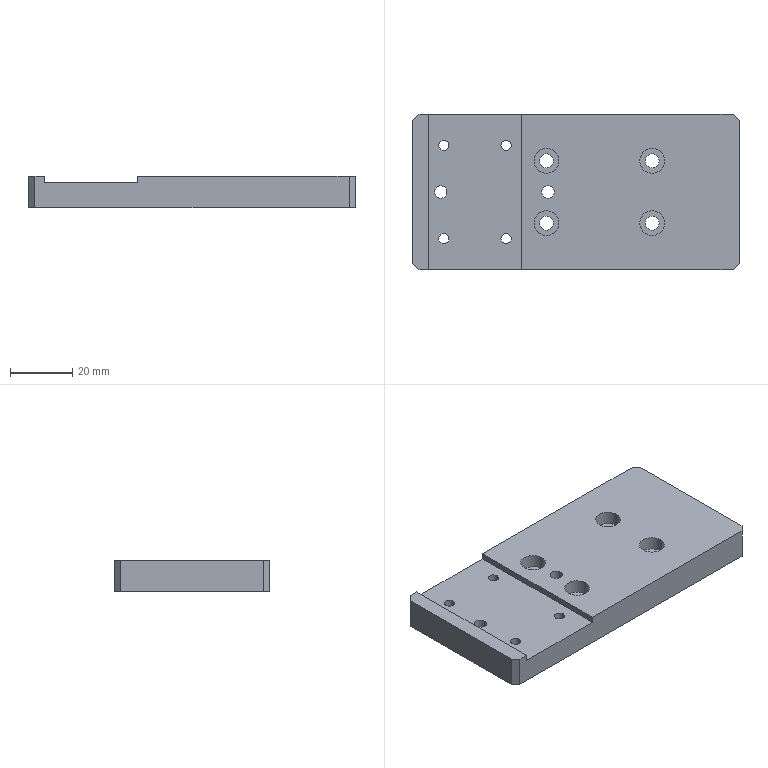Part | SolidWorks | mm | material S45C | 1 solid | 46 faces | box 105 x 50 x 10 mm | volume 47679 mm3 | cylinder 28 | plane 18 | commonest cylinder face diameters 3.3 x8 8 x8 4.5 x8 4 x4
Drawing notes:
C2.0 TYP ALL 4 CORNERS (TOP VIEW) | from the solid: Plate bbox 105.0 x 50.0 x 10.0; outline planes x=0/105, y=0/50 with all four plan corners broken identically; only chamfer size given on drawing is C2.0, no cones/fillets listed
2X Ø4.00 +0.01/+0.02 THRU @ X9.00 & X43.50, Y25.00 | from the solid: Ø4.0 z-axis holes at (9.0,25.0) and (43.5,25.0); dims from 0,0 corner used by drawing
build123d program:
from build123d import *

# Parameters (mm, degrees)
SKETCH1_W                                       = 105
SKETCH1_H                                       = 50
BOSS_EXTRUDE1_DEPTH                             = 10
SKETCH2_W                                       = 30
SKETCH2_H                                       = 50
CUT_EXTRUDE1_DEPTH                              = 2
M4_HEX_SOCKET_HEAD_CAP_SCREW_CBORE1_D           = 4.5
M4_HEX_SOCKET_HEAD_CAP_SCREW_CBORE1_CBORE_D     = 8
M4_HEX_SOCKET_HEAD_CAP_SCREW_CBORE1_CBORE_DEPTH = 4.4
SIZE_MM_DOWEL_PIN_HOLE1_D                       = 4
M4_TAPPED_HOLE1_D                               = 3.3
CHAMFER1_SIZE                                   = 2


with BuildPart() as part:
    # Sketch1 → Boss-Extrude1 (new body)
    with BuildSketch(Plane.XY):
        Rectangle(SKETCH1_W, SKETCH1_H)
    extrude(amount=BOSS_EXTRUDE1_DEPTH)

    # Sketch2 → Cut-Extrude1 (cut)
    with BuildSketch(Plane.XY.offset(10)):
        with Locations((-32.5, 0)):
            Rectangle(SKETCH2_W, SKETCH2_H)
    extrude(amount=-CUT_EXTRUDE1_DEPTH, mode=Mode.SUBTRACT)

    # M4 Hex Socket Head Cap Screw CBORE1 (through all)
    with Locations(Plane.XY.offset(10)):
        with Locations((-9.5, 10), (24.5, 10), (24.5, -10), (-9.5, -10)):
            CounterBoreHole(M4_HEX_SOCKET_HEAD_CAP_SCREW_CBORE1_D / 2, M4_HEX_SOCKET_HEAD_CAP_SCREW_CBORE1_CBORE_D / 2, M4_HEX_SOCKET_HEAD_CAP_SCREW_CBORE1_CBORE_DEPTH)

    # Size mm Dowel Pin Hole1 (through all)
    with Locations(Plane.XY.offset(10)):
        with Locations((-9, 0), (-43.5, 0)):
            Hole(SIZE_MM_DOWEL_PIN_HOLE1_D / 2)

    # M4 Tapped Hole1 (through all)
    with Locations(Plane.XY.offset(8)):
        with Locations((-42.5, 15), (-22.5, 15), (-22.5, -15), (-42.5, -15)):
            Hole(M4_TAPPED_HOLE1_D / 2)

    # Chamfer1
    chamfer1_edges = [part.edges().sort_by_distance(p)[0] for p in [
        (52.5, -25, 5),
        (-52.5, -25, 5),
        (-52.5, 25, 5),
        (52.5, 25, 5),
    ]]
    chamfer(chamfer1_edges, length=CHAMFER1_SIZE)


solid = part.part